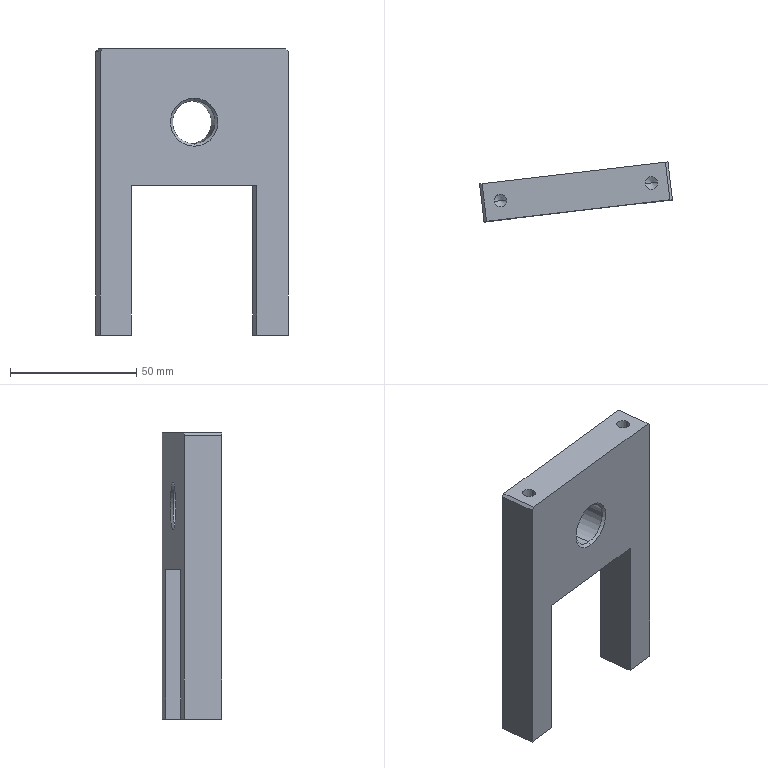Component | SolidWorks | 8TC-A17001-90-02PressureRollerSidePlate2-1 | 1 solid | 34 faces | box 76.24 x 23.65 x 113.2 mm | volume 77668 mm3 | cone 12 | plane 12 | cylinder 10 | commonest cylinder face diameters 5 x8 17 x2 | material #45
build123d program:
from build123d import *

# Parameters (mm, degrees)
SKETCH1_W                  = 75
SKETCH1_H                  = 54
BOSS_EXTRUDE1_DEPTH        = 7.5
SKETCH23_W                 = 12.5
SKETCH23_H                 = 15
BOSS_EXTRUDE4_DEPTH        = 59.2
M6_TAPPED_HOLE2_D          = 5
M6_TAPPED_HOLE2_DEPTH      = 25
M6_TAPPED_HOLE2_TIP        = 1.502
M6_TAPPED_HOLE1_D          = 5
M6_TAPPED_HOLE1_DEPTH      = 20
M6_TAPPED_HOLE1_TIP        = 1.502
F_15_0_15_DIAMETER_HOLE1_D = 17
CHAMFER2_SIZE              = 1


with BuildPart() as part:
    # Sketch1 → Boss-Extrude1 (new, symmetric)
    with BuildSketch(Plane(origin=(0, 0, 0), x_dir=(1, 0, 0), z_dir=(0, 1, 0))):
        Rectangle(SKETCH1_W, SKETCH1_H)
    extrude(amount=BOSS_EXTRUDE1_DEPTH, both=True)

    # Sketch23 → Boss-Extrude4 (add)
    with BuildSketch(Plane.XY.offset(27)):
        with Locations((-31.25, 0)):
            Rectangle(SKETCH23_W, SKETCH23_H)
        with Locations((31.25, 0)):
            Rectangle(SKETCH23_W, SKETCH23_H)
    extrude(amount=BOSS_EXTRUDE4_DEPTH)

    # M6 Tapped Hole2
    with Locations(Plane.XY.offset(86.2)):
        with Locations((-30, 0), (30, 0)):
            Hole(M6_TAPPED_HOLE2_D / 2, depth=M6_TAPPED_HOLE2_DEPTH)
            with Locations((0, 0, -(M6_TAPPED_HOLE2_DEPTH + M6_TAPPED_HOLE2_TIP / 2))):  # 118° drill point
                Cone(0, M6_TAPPED_HOLE2_D / 2, M6_TAPPED_HOLE2_TIP, mode=Mode.SUBTRACT)

    # M6 Tapped Hole1
    with Locations(Plane(origin=(0, 0, -27), x_dir=(-1, 0, 0), z_dir=(0, 0, -1))):
        with Locations((-30, 0), (30, 0)):
            Hole(M6_TAPPED_HOLE1_D / 2, depth=M6_TAPPED_HOLE1_DEPTH)
            with Locations((0, 0, -(M6_TAPPED_HOLE1_DEPTH + M6_TAPPED_HOLE1_TIP / 2))):  # 118° drill point
                Cone(0, M6_TAPPED_HOLE1_D / 2, M6_TAPPED_HOLE1_TIP, mode=Mode.SUBTRACT)

    # 15.0 _15_ Diameter Hole1 (through all)
    with Locations(Plane(origin=(0, 7.5, 0), x_dir=(1, 0, 0), z_dir=(0, 1, 0))):
        with Locations((0, -2)):
            Hole(F_15_0_15_DIAMETER_HOLE1_D / 2)

    # Chamfer2
    chamfer2_edges = [part.edges().sort_by_distance(p)[0] for p in [
        (8.5, -7.5, 2),
        (8.5, 7.5, 2),
        (-37.5, 0, -27),
        (37.5, 0, -27),
    ]]
    chamfer(chamfer2_edges, length=CHAMFER2_SIZE)


solid = part.part

# Placed as in the assembly
solid = solid.moved(Location((-0.2049, 42.224, -50), (180, 0, 173.3)))
STEP:
#1=COLOUR_RGB('',0.7922,0.8196,0.9333);
#2=FILL_AREA_STYLE_COLOUR('',#1);
#3=FILL_AREA_STYLE('',(#2));
#4=SURFACE_STYLE_FILL_AREA(#3);
#5=SURFACE_SIDE_STYLE('',(#4));
#6=SURFACE_STYLE_USAGE(.BOTH.,#5);
#7=PRESENTATION_STYLE_ASSIGNMENT((#6));
#8=CARTESIAN_POINT('',(-0.03792,1.917,-1.713));
#9=VERTEX_POINT('',#8);
#10=CARTESIAN_POINT('',(-0.03792,1.917,-2.382));
#11=VERTEX_POINT('',#10);
#12=CARTESIAN_POINT('',(-0.03792,1.917,-2.047));
#13=DIRECTION('',(-0.1167,0.9932,0.));
#14=DIRECTION('',(-0.,0.,-1.));
#15=AXIS2_PLACEMENT_3D('',#12,#13,#14);
#16=CIRCLE('',#15,0.3346);
#17=EDGE_CURVE('',#9,#11,#16,.T.);
#18=ORIENTED_EDGE('',*,*,#17,.F.);
#19=CARTESIAN_POINT('',(-0.04251,1.956,-1.673));
#20=VERTEX_POINT('',#19);
#21=CARTESIAN_POINT('',(-0.03792,1.917,-1.713));
#22=DIRECTION('',(-0.0825,0.7023,0.7071));
#23=VECTOR('',#22,39.37);
#24=LINE('',#21,#23);
#25=EDGE_CURVE('',#9,#20,#24,.T.);
#26=ORIENTED_EDGE('',*,*,#25,.T.);
#27=CARTESIAN_POINT('',(-0.04251,1.956,-2.421));
#28=VERTEX_POINT('',#27);
#29=CARTESIAN_POINT('',(-0.04251,1.956,-2.047));
#30=DIRECTION('',(0.1167,-0.9932,-0.));
#31=DIRECTION('',(-0.,0.,-1.));
#32=AXIS2_PLACEMENT_3D('',#29,#30,#31);
#33=CIRCLE('',#32,0.374);
#34=EDGE_CURVE('',#28,#20,#33,.T.);
#35=ORIENTED_EDGE('',*,*,#34,.F.);
#36=CARTESIAN_POINT('',(-0.03792,1.917,-2.382));
#37=DIRECTION('',(-0.0825,0.7023,-0.7071));
#38=VECTOR('',#37,39.37);
#39=LINE('',#36,#38);
#40=EDGE_CURVE('',#11,#28,#39,.T.);
#41=ORIENTED_EDGE('',*,*,#40,.F.);
#42=EDGE_LOOP('',(#18,#26,#35,#41));
#43=FACE_OUTER_BOUND('',#42,.T.);
#44=CARTESIAN_POINT('',(-0.03792,1.917,-2.047));
#45=DIRECTION('',(-0.1167,0.9932,0.));
#46=DIRECTION('',(-0.,0.,-1.));
#47=AXIS2_PLACEMENT_3D('',#44,#45,#46);
#48=CONICAL_SURFACE('',#47,0.3346,0.7854);
#49=ADVANCED_FACE('',(#43),#48,.F.);
#50=CARTESIAN_POINT('',(0.02179,1.408,-2.382));
#51=VERTEX_POINT('',#50);
#52=CARTESIAN_POINT('',(0.02179,1.408,-1.713));
#53=VERTEX_POINT('',#52);
#54=CARTESIAN_POINT('',(0.02179,1.408,-2.047));
#55=DIRECTION('',(0.1167,-0.9932,-0.));
#56=DIRECTION('',(-0.,0.,-1.));
#57=AXIS2_PLACEMENT_3D('',#54,#55,#56);
#58=CIRCLE('',#57,0.3346);
#59=EDGE_CURVE('',#51,#53,#58,.T.);
#60=ORIENTED_EDGE('',*,*,#59,.F.);
#61=CARTESIAN_POINT('',(0.02638,1.369,-2.421));
#62=VERTEX_POINT('',#61);
#63=CARTESIAN_POINT('',(0.02638,1.369,-2.421));
#64=DIRECTION('',(0.0825,-0.7023,-0.7071));
#65=VECTOR('',#64,39.37);
#66=LINE('',#63,#65);
#67=EDGE_CURVE('',#51,#62,#66,.T.);
#68=ORIENTED_EDGE('',*,*,#67,.T.);
#69=CARTESIAN_POINT('',(0.02638,1.369,-1.673));
#70=VERTEX_POINT('',#69);
#71=CARTESIAN_POINT('',(0.02638,1.369,-2.047));
#72=DIRECTION('',(-0.1167,0.9932,0.));
#73=DIRECTION('',(-0.,0.,-1.));
#74=AXIS2_PLACEMENT_3D('',#71,#72,#73);
#75=CIRCLE('',#74,0.374);
#76=EDGE_CURVE('',#70,#62,#75,.T.);
#77=ORIENTED_EDGE('',*,*,#76,.F.);
#78=CARTESIAN_POINT('',(0.02638,1.369,-1.673));
#79=DIRECTION('',(0.0825,-0.7023,0.7071));
#80=VECTOR('',#79,39.37);
#81=LINE('',#78,#80);
#82=EDGE_CURVE('',#53,#70,#81,.T.);
#83=ORIENTED_EDGE('',*,*,#82,.F.);
#84=EDGE_LOOP('',(#60,#68,#77,#83));
#85=FACE_OUTER_BOUND('',#84,.T.);
#86=CARTESIAN_POINT('',(0.02638,1.369,-2.047));
#87=DIRECTION('',(0.1167,-0.9932,-0.));
#88=DIRECTION('',(0.,0.,1.));
#89=AXIS2_PLACEMENT_3D('',#86,#87,#88);
#90=CONICAL_SURFACE('',#89,0.374,0.7854);
#91=ADVANCED_FACE('',(#85),#90,.F.);
#92=ORIENTED_EDGE('',*,*,#59,.T.);
#93=CARTESIAN_POINT('',(-0.04251,1.956,-1.713));
#94=DIRECTION('',(-0.1167,0.9932,0.));
#95=VECTOR('',#94,39.37);
#96=LINE('',#93,#95);
#97=EDGE_CURVE('',#53,#9,#96,.T.);
#98=ORIENTED_EDGE('',*,*,#97,.T.);
#99=ORIENTED_EDGE('',*,*,#17,.T.);
#100=CARTESIAN_POINT('',(-0.04251,1.956,-2.382));
#101=DIRECTION('',(-0.1167,0.9932,0.));
#102=VECTOR('',#101,39.37);
#103=LINE('',#100,#102);
#104=EDGE_CURVE('',#51,#11,#103,.T.);
#105=ORIENTED_EDGE('',*,*,#104,.F.);
#106=EDGE_LOOP('',(#92,#98,#99,#105));
#107=FACE_OUTER_BOUND('',#106,.T.);
#108=CARTESIAN_POINT('',(-0.04251,1.956,-2.047));
#109=DIRECTION('',(-0.1167,0.9932,0.));
#110=DIRECTION('',(-0.,0.,-1.));
#111=AXIS2_PLACEMENT_3D('',#108,#109,#110);
#112=CYLINDRICAL_SURFACE('',#111,0.3346);
#113=ADVANCED_FACE('',(#107),#112,.F.);
#114=CARTESIAN_POINT('',(-1.279,1.513,-1.693));
#115=VERTEX_POINT('',#114);
#116=CARTESIAN_POINT('',(-1.083,1.536,-1.693));
#117=VERTEX_POINT('',#116);
#118=CARTESIAN_POINT('',(-1.181,1.525,-1.693));
#119=DIRECTION('',(0.,-0.,1.));
#120=DIRECTION('',(0.9932,0.1167,0.));
#121=AXIS2_PLACEMENT_3D('',#118,#119,#120);
#122=CIRCLE('',#121,0.09843);
#123=EDGE_CURVE('',#115,#117,#122,.T.);
#124=ORIENTED_EDGE('',*,*,#123,.F.);
#125=CARTESIAN_POINT('',(-1.279,1.513,-0.9055));
#126=VERTEX_POINT('',#125);
#127=CARTESIAN_POINT('',(-1.279,1.513,-0.9055));
#128=DIRECTION('',(0.,-0.,1.));
#129=VECTOR('',#128,39.37);
#130=LINE('',#127,#129);
#131=EDGE_CURVE('',#115,#126,#130,.T.);
#132=ORIENTED_EDGE('',*,*,#131,.T.);
#133=CARTESIAN_POINT('',(-1.083,1.536,-0.9055));
#134=VERTEX_POINT('',#133);
#135=CARTESIAN_POINT('',(-1.181,1.525,-0.9055));
#136=DIRECTION('',(0.,-0.,1.));
#137=DIRECTION('',(0.9932,0.1167,0.));
#138=AXIS2_PLACEMENT_3D('',#135,#136,#137);
#139=CIRCLE('',#138,0.09843);
#140=EDGE_CURVE('',#126,#134,#139,.T.);
#141=ORIENTED_EDGE('',*,*,#140,.T.);
#142=CARTESIAN_POINT('',(-1.083,1.536,-0.9055));
#143=DIRECTION('',(0.,-0.,1.));
#144=VECTOR('',#143,39.37);
#145=LINE('',#142,#144);
#146=EDGE_CURVE('',#117,#134,#145,.T.);
#147=ORIENTED_EDGE('',*,*,#146,.F.);
#148=EDGE_LOOP('',(#124,#132,#141,#147));
#149=FACE_OUTER_BOUND('',#148,.T.);
#150=CARTESIAN_POINT('',(-1.181,1.525,-0.9055));
#151=DIRECTION('',(0.,-0.,1.));
#152=DIRECTION('',(0.9932,0.1167,0.));
#153=AXIS2_PLACEMENT_3D('',#150,#151,#152);
#154=CYLINDRICAL_SURFACE('',#153,0.09843);
#155=ADVANCED_FACE('',(#149),#154,.F.);
#156=CARTESIAN_POINT('',(-1.181,1.525,-1.752));
#157=VERTEX_POINT('',#156);
#158=CARTESIAN_POINT('',(-1.083,1.536,-1.693));
#159=DIRECTION('',(0.8513,0.1,0.515));
#160=VECTOR('',#159,39.37);
#161=LINE('',#158,#160);
#162=EDGE_CURVE('',#157,#117,#161,.T.);
#163=ORIENTED_EDGE('',*,*,#162,.F.);
#164=CARTESIAN_POINT('',(-1.279,1.513,-1.693));
#165=DIRECTION('',(-0.8513,-0.1,0.515));
#166=VECTOR('',#165,39.37);
#167=LINE('',#164,#166);
#168=EDGE_CURVE('',#157,#115,#167,.T.);
#169=ORIENTED_EDGE('',*,*,#168,.T.);
#170=ORIENTED_EDGE('',*,*,#123,.T.);
#171=EDGE_LOOP('',(#163,#169,#170));
#172=FACE_OUTER_BOUND('',#171,.T.);
#173=CARTESIAN_POINT('',(-1.181,1.525,-1.693));
#174=DIRECTION('',(0.,-0.,1.));
#175=DIRECTION('',(0.9932,0.1167,0.));
#176=AXIS2_PLACEMENT_3D('',#173,#174,#175);
#177=CONICAL_SURFACE('',#176,0.09843,1.03);
#178=ADVANCED_FACE('',(#172),#177,.F.);
#179=CARTESIAN_POINT('',(1.067,1.789,-1.693));
#180=VERTEX_POINT('',#179);
#181=CARTESIAN_POINT('',(1.263,1.812,-1.693));
#182=VERTEX_POINT('',#181);
#183=CARTESIAN_POINT('',(1.165,1.8,-1.693));
#184=DIRECTION('',(0.,-0.,1.));
#185=DIRECTION('',(0.9932,0.1167,0.));
#186=AXIS2_PLACEMENT_3D('',#183,#184,#185);
#187=CIRCLE('',#186,0.09843);
#188=EDGE_CURVE('',#180,#182,#187,.T.);
#189=ORIENTED_EDGE('',*,*,#188,.F.);
#190=CARTESIAN_POINT('',(1.067,1.789,-0.9055));
#191=VERTEX_POINT('',#190);
#192=CARTESIAN_POINT('',(1.067,1.789,-0.9055));
#193=DIRECTION('',(0.,-0.,1.));
#194=VECTOR('',#193,39.37);
#195=LINE('',#192,#194);
#196=EDGE_CURVE('',#180,#191,#195,.T.);
#197=ORIENTED_EDGE('',*,*,#196,.T.);
#198=CARTESIAN_POINT('',(1.263,1.812,-0.9055));
#199=VERTEX_POINT('',#198);
#200=CARTESIAN_POINT('',(1.165,1.8,-0.9055));
#201=DIRECTION('',(0.,-0.,1.));
#202=DIRECTION('',(0.9932,0.1167,0.));
#203=AXIS2_PLACEMENT_3D('',#200,#201,#202);
#204=CIRCLE('',#203,0.09843);
#205=EDGE_CURVE('',#191,#199,#204,.T.);
#206=ORIENTED_EDGE('',*,*,#205,.T.);
#207=CARTESIAN_POINT('',(1.263,1.812,-0.9055));
#208=DIRECTION('',(0.,-0.,1.));
#209=VECTOR('',#208,39.37);
#210=LINE('',#207,#209);
#211=EDGE_CURVE('',#182,#199,#210,.T.);
#212=ORIENTED_EDGE('',*,*,#211,.F.);
#213=EDGE_LOOP('',(#189,#197,#206,#212));
#214=FACE_OUTER_BOUND('',#213,.T.);
#215=CARTESIAN_POINT('',(1.165,1.8,-0.9055));
#216=DIRECTION('',(0.,-0.,1.));
#217=DIRECTION('',(0.9932,0.1167,0.));
#218=AXIS2_PLACEMENT_3D('',#215,#216,#217);
#219=CYLINDRICAL_SURFACE('',#218,0.09843);
#220=ADVANCED_FACE('',(#214),#219,.F.);
#221=CARTESIAN_POINT('',(1.165,1.8,-1.752));
#222=VERTEX_POINT('',#221);
#223=CARTESIAN_POINT('',(1.263,1.812,-1.693));
#224=DIRECTION('',(0.8513,0.1,0.515));
#225=VECTOR('',#224,39.37);
#226=LINE('',#223,#225);
#227=EDGE_CURVE('',#222,#182,#226,.T.);
#228=ORIENTED_EDGE('',*,*,#227,.F.);
#229=CARTESIAN_POINT('',(1.067,1.789,-1.693));
#230=DIRECTION('',(-0.8513,-0.1,0.515));
#231=VECTOR('',#230,39.37);
#232=LINE('',#229,#231);
#233=EDGE_CURVE('',#222,#180,#232,.T.);
#234=ORIENTED_EDGE('',*,*,#233,.T.);
#235=ORIENTED_EDGE('',*,*,#188,.T.);
#236=EDGE_LOOP('',(#228,#234,#235));
#237=FACE_OUTER_BOUND('',#236,.T.);
#238=CARTESIAN_POINT('',(1.165,1.8,-1.693));
#239=DIRECTION('',(0.,-0.,1.));
#240=DIRECTION('',(0.9932,0.1167,0.));
#241=AXIS2_PLACEMENT_3D('',#238,#239,#240);
#242=CONICAL_SURFACE('',#241,0.09843,1.03);
#243=ADVANCED_FACE('',(#237),#242,.F.);
#244=CARTESIAN_POINT('',(1.263,1.812,-4.378));
#245=VERTEX_POINT('',#244);
#246=CARTESIAN_POINT('',(1.067,1.789,-4.378));
#247=VERTEX_POINT('',#246);
#248=CARTESIAN_POINT('',(1.165,1.8,-4.378));
#249=DIRECTION('',(-0.,0.,-1.));
#250=DIRECTION('',(-0.9932,-0.1167,0.));
#251=AXIS2_PLACEMENT_3D('',#248,#249,#250);
#252=CIRCLE('',#251,0.09843);
#253=EDGE_CURVE('',#245,#247,#252,.T.);
#254=ORIENTED_EDGE('',*,*,#253,.F.);
#255=CARTESIAN_POINT('',(1.263,1.812,-5.362));
#256=VERTEX_POINT('',#255);
#257=CARTESIAN_POINT('',(1.263,1.812,-5.362));
#258=DIRECTION('',(-0.,0.,-1.));
#259=VECTOR('',#258,39.37);
#260=LINE('',#257,#259);
#261=EDGE_CURVE('',#245,#256,#260,.T.);
#262=ORIENTED_EDGE('',*,*,#261,.T.);
#263=CARTESIAN_POINT('',(1.067,1.789,-5.362));
#264=VERTEX_POINT('',#263);
#265=CARTESIAN_POINT('',(1.165,1.8,-5.362));
#266=DIRECTION('',(-0.,0.,-1.));
#267=DIRECTION('',(-0.9932,-0.1167,0.));
#268=AXIS2_PLACEMENT_3D('',#265,#266,#267);
#269=CIRCLE('',#268,0.09843);
#270=EDGE_CURVE('',#256,#264,#269,.T.);
#271=ORIENTED_EDGE('',*,*,#270,.T.);
#272=CARTESIAN_POINT('',(1.067,1.789,-5.362));
#273=DIRECTION('',(-0.,0.,-1.));
#274=VECTOR('',#273,39.37);
#275=LINE('',#272,#274);
#276=EDGE_CURVE('',#247,#264,#275,.T.);
#277=ORIENTED_EDGE('',*,*,#276,.F.);
#278=EDGE_LOOP('',(#254,#262,#271,#277));
#279=FACE_OUTER_BOUND('',#278,.T.);
#280=CARTESIAN_POINT('',(1.165,1.8,-5.362));
#281=DIRECTION('',(-0.,0.,-1.));
#282=DIRECTION('',(-0.9932,-0.1167,0.));
#283=AXIS2_PLACEMENT_3D('',#280,#281,#282);
#284=CYLINDRICAL_SURFACE('',#283,0.09843);
#285=ADVANCED_FACE('',(#279),#284,.F.);
#286=CARTESIAN_POINT('',(1.165,1.8,-4.319));
#287=VERTEX_POINT('',#286);
#288=CARTESIAN_POINT('',(1.067,1.789,-4.378));
#289=DIRECTION('',(-0.8513,-0.1,-0.515));
#290=VECTOR('',#289,39.37);
#291=LINE('',#288,#290);
#292=EDGE_CURVE('',#287,#247,#291,.T.);
#293=ORIENTED_EDGE('',*,*,#292,.F.);
#294=CARTESIAN_POINT('',(1.263,1.812,-4.378));
#295=DIRECTION('',(0.8513,0.1,-0.515));
#296=VECTOR('',#295,39.37);
#297=LINE('',#294,#296);
#298=EDGE_CURVE('',#287,#245,#297,.T.);
#299=ORIENTED_EDGE('',*,*,#298,.T.);
#300=ORIENTED_EDGE('',*,*,#253,.T.);
#301=EDGE_LOOP('',(#293,#299,#300));
#302=FACE_OUTER_BOUND('',#301,.T.);
#303=CARTESIAN_POINT('',(1.165,1.8,-4.378));
#304=DIRECTION('',(-0.,0.,-1.));
#305=DIRECTION('',(-0.9932,-0.1167,0.));
#306=AXIS2_PLACEMENT_3D('',#303,#304,#305);
#307=CONICAL_SURFACE('',#306,0.09843,1.03);
#308=ADVANCED_FACE('',(#302),#307,.F.);
#309=CARTESIAN_POINT('',(-1.083,1.536,-4.378));
#310=VERTEX_POINT('',#309);
#311=CARTESIAN_POINT('',(-1.279,1.513,-4.378));
#312=VERTEX_POINT('',#311);
#313=CARTESIAN_POINT('',(-1.181,1.525,-4.378));
#314=DIRECTION('',(-0.,0.,-1.));
#315=DIRECTION('',(-0.9932,-0.1167,0.));
#316=AXIS2_PLACEMENT_3D('',#313,#314,#315);
#317=CIRCLE('',#316,0.09843);
#318=EDGE_CURVE('',#310,#312,#317,.T.);
#319=ORIENTED_EDGE('',*,*,#318,.F.);
#320=CARTESIAN_POINT('',(-1.083,1.536,-5.362));
#321=VERTEX_POINT('',#320);
#322=CARTESIAN_POINT('',(-1.083,1.536,-5.362));
#323=DIRECTION('',(-0.,0.,-1.));
#324=VECTOR('',#323,39.37);
#325=LINE('',#322,#324);
#326=EDGE_CURVE('',#310,#321,#325,.T.);
#327=ORIENTED_EDGE('',*,*,#326,.T.);
#328=CARTESIAN_POINT('',(-1.279,1.513,-5.362));
#329=VERTEX_POINT('',#328);
#330=CARTESIAN_POINT('',(-1.181,1.525,-5.362));
#331=DIRECTION('',(-0.,0.,-1.));
#332=DIRECTION('',(-0.9932,-0.1167,0.));
#333=AXIS2_PLACEMENT_3D('',#330,#331,#332);
#334=CIRCLE('',#333,0.09843);
#335=EDGE_CURVE('',#321,#329,#334,.T.);
#336=ORIENTED_EDGE('',*,*,#335,.T.);
#337=CARTESIAN_POINT('',(-1.279,1.513,-5.362));
#338=DIRECTION('',(-0.,0.,-1.));
#339=VECTOR('',#338,39.37);
#340=LINE('',#337,#339);
#341=EDGE_CURVE('',#312,#329,#340,.T.);
#342=ORIENTED_EDGE('',*,*,#341,.F.);
#343=EDGE_LOOP('',(#319,#327,#336,#342));
#344=FACE_OUTER_BOUND('',#343,.T.);
#345=CARTESIAN_POINT('',(-1.181,1.525,-5.362));
#346=DIRECTION('',(-0.,0.,-1.));
#347=DIRECTION('',(-0.9932,-0.1167,0.));
#348=AXIS2_PLACEMENT_3D('',#345,#346,#347);
#349=CYLINDRICAL_SURFACE('',#348,0.09843);
#350=ADVANCED_FACE('',(#344),#349,.F.);
#351=CARTESIAN_POINT('',(-1.181,1.525,-4.319));
#352=VERTEX_POINT('',#351);
#353=CARTESIAN_POINT('',(-1.279,1.513,-4.378));
#354=DIRECTION('',(-0.8513,-0.1,-0.515));
#355=VECTOR('',#354,39.37);
#356=LINE('',#353,#355);
#357=EDGE_CURVE('',#352,#312,#356,.T.);
#358=ORIENTED_EDGE('',*,*,#357,.F.);
#359=CARTESIAN_POINT('',(-1.083,1.536,-4.378));
#360=DIRECTION('',(0.8513,0.1,-0.515));
#361=VECTOR('',#360,39.37);
#362=LINE('',#359,#361);
#363=EDGE_CURVE('',#352,#310,#362,.T.);
#364=ORIENTED_EDGE('',*,*,#363,.T.);
#365=ORIENTED_EDGE('',*,*,#318,.T.);
#366=EDGE_LOOP('',(#358,#364,#365));
#367=FACE_OUTER_BOUND('',#366,.T.);
#368=CARTESIAN_POINT('',(-1.181,1.525,-4.378));
#369=DIRECTION('',(-0.,0.,-1.));
#370=DIRECTION('',(-0.9932,-0.1167,0.));
#371=AXIS2_PLACEMENT_3D('',#368,#369,#370);
#372=CONICAL_SURFACE('',#371,0.09843,1.03);
#373=ADVANCED_FACE('',(#367),#372,.F.);
#374=CARTESIAN_POINT('',(-1.02,1.841,-3.031));
#375=VERTEX_POINT('',#374);
#376=CARTESIAN_POINT('',(-0.9511,1.254,-3.031));
#377=VERTEX_POINT('',#376);
#378=CARTESIAN_POINT('',(-1.02,1.841,-3.031));
#379=DIRECTION('',(0.1167,-0.9932,-0.));
#380=VECTOR('',#379,39.37);
#381=LINE('',#378,#380);
#382=EDGE_CURVE('',#375,#377,#381,.T.);
#383=ORIENTED_EDGE('',*,*,#382,.F.);
#384=CARTESIAN_POINT('',(0.935,2.07,-3.031));
#385=VERTEX_POINT('',#384);
#386=CARTESIAN_POINT('',(1.424,2.128,-3.031));
#387=DIRECTION('',(-0.9932,-0.1167,0.));
#388=VECTOR('',#387,39.37);
#389=LINE('',#386,#388);
#390=EDGE_CURVE('',#385,#375,#389,.T.);
#391=ORIENTED_EDGE('',*,*,#390,.F.);
#392=CARTESIAN_POINT('',(1.004,1.484,-3.031));
#393=VERTEX_POINT('',#392);
#394=CARTESIAN_POINT('',(0.935,2.07,-3.031));
#395=DIRECTION('',(-0.1167,0.9932,0.));
#396=VECTOR('',#395,39.37);
#397=LINE('',#394,#396);
#398=EDGE_CURVE('',#393,#385,#397,.T.);
#399=ORIENTED_EDGE('',*,*,#398,.F.);
#400=CARTESIAN_POINT('',(1.493,1.541,-3.031));
#401=DIRECTION('',(-0.9932,-0.1167,0.));
#402=VECTOR('',#401,39.37);
#403=LINE('',#400,#402);
#404=EDGE_CURVE('',#393,#377,#403,.T.);
#405=ORIENTED_EDGE('',*,*,#404,.T.);
#406=EDGE_LOOP('',(#383,#391,#399,#405));
#407=FACE_OUTER_BOUND('',#406,.T.);
#408=CARTESIAN_POINT('',(1.424,2.128,-3.031));
#409=DIRECTION('',(0.,-0.,1.));
#410=DIRECTION('',(0.9932,0.1167,-0.));
#411=AXIS2_PLACEMENT_3D('',#408,#409,#410);
#412=PLANE('',#411);
#413=ADVANCED_FACE('',(#407),#412,.F.);
#414=CARTESIAN_POINT('',(-1.44,1.197,-5.362));
#415=VERTEX_POINT('',#414);
#416=CARTESIAN_POINT('',(-1.44,1.197,-0.9449));
#417=VERTEX_POINT('',#416);
#418=CARTESIAN_POINT('',(-1.44,1.197,-0.9055));
#419=DIRECTION('',(0.,-0.,1.));
#420=VECTOR('',#419,39.37);
#421=LINE('',#418,#420);
#422=EDGE_CURVE('',#415,#417,#421,.T.);
#423=ORIENTED_EDGE('',*,*,#422,.T.);
#424=CARTESIAN_POINT('',(-1.509,1.783,-0.9449));
#425=VERTEX_POINT('',#424);
#426=CARTESIAN_POINT('',(-1.509,1.783,-0.9449));
#427=DIRECTION('',(-0.1167,0.9932,0.));
#428=VECTOR('',#427,39.37);
#429=LINE('',#426,#428);
#430=EDGE_CURVE('',#417,#425,#429,.T.);
#431=ORIENTED_EDGE('',*,*,#430,.T.);
#432=CARTESIAN_POINT('',(-1.509,1.783,-5.362));
#433=VERTEX_POINT('',#432);
#434=CARTESIAN_POINT('',(-1.509,1.783,-0.9055));
#435=DIRECTION('',(0.,-0.,1.));
#436=VECTOR('',#435,39.37);
#437=LINE('',#434,#436);
#438=EDGE_CURVE('',#433,#425,#437,.T.);
#439=ORIENTED_EDGE('',*,*,#438,.F.);
#440=CARTESIAN_POINT('',(-1.509,1.783,-5.362));
#441=DIRECTION('',(-0.1167,0.9932,0.));
#442=VECTOR('',#441,39.37);
#443=LINE('',#440,#442);
#444=EDGE_CURVE('',#415,#433,#443,.T.);
#445=ORIENTED_EDGE('',*,*,#444,.F.);
#446=EDGE_LOOP('',(#423,#431,#439,#445));
#447=FACE_OUTER_BOUND('',#446,.T.);
#448=CARTESIAN_POINT('',(-1.509,1.783,-0.9055));
#449=DIRECTION('',(0.9932,0.1167,-0.));
#450=DIRECTION('',(-0.,0.,-1.));
#451=AXIS2_PLACEMENT_3D('',#448,#449,#450);
#452=PLANE('',#451);
#453=ADVANCED_FACE('',(#447),#452,.F.);
#454=CARTESIAN_POINT('',(-1.181,1.525,-0.9055));
#455=DIRECTION('',(0.,-0.,1.));
#456=DIRECTION('',(0.9932,0.1167,0.));
#457=AXIS2_PLACEMENT_3D('',#454,#455,#456);
#458=CIRCLE('',#457,0.09843);
#459=EDGE_CURVE('',#134,#126,#458,.T.);
#460=ORIENTED_EDGE('',*,*,#459,.F.);
#461=ORIENTED_EDGE('',*,*,#140,.F.);
#462=EDGE_LOOP('',(#460,#461));
#463=FACE_BOUND('',#462,.T.);
#464=CARTESIAN_POINT('',(1.165,1.8,-0.9055));
#465=DIRECTION('',(0.,-0.,1.));
#466=DIRECTION('',(0.9932,0.1167,0.));
#467=AXIS2_PLACEMENT_3D('',#464,#465,#466);
#468=CIRCLE('',#467,0.09843);
#469=EDGE_CURVE('',#199,#191,#468,.T.);
#470=ORIENTED_EDGE('',*,*,#469,.F.);
#471=ORIENTED_EDGE('',*,*,#205,.F.);
#472=EDGE_LOOP('',(#470,#471));
#473=FACE_BOUND('',#472,.T.);
#474=CARTESIAN_POINT('',(-1.401,1.201,-0.9055));
#475=VERTEX_POINT('',#474);
#476=CARTESIAN_POINT('',(1.454,1.537,-0.9055));
#477=VERTEX_POINT('',#476);
#478=CARTESIAN_POINT('',(1.493,1.541,-0.9055));
#479=DIRECTION('',(0.9932,0.1167,-0.));
#480=VECTOR('',#479,39.37);
#481=LINE('',#478,#480);
#482=EDGE_CURVE('',#475,#477,#481,.T.);
#483=ORIENTED_EDGE('',*,*,#482,.T.);
#484=CARTESIAN_POINT('',(1.385,2.123,-0.9055));
#485=VERTEX_POINT('',#484);
#486=CARTESIAN_POINT('',(1.385,2.123,-0.9055));
#487=DIRECTION('',(-0.1167,0.9932,0.));
#488=VECTOR('',#487,39.37);
#489=LINE('',#486,#488);
#490=EDGE_CURVE('',#477,#485,#489,.T.);
#491=ORIENTED_EDGE('',*,*,#490,.T.);
#492=CARTESIAN_POINT('',(-1.47,1.788,-0.9055));
#493=VERTEX_POINT('',#492);
#494=CARTESIAN_POINT('',(1.424,2.128,-0.9055));
#495=DIRECTION('',(0.9932,0.1167,-0.));
#496=VECTOR('',#495,39.37);
#497=LINE('',#494,#496);
#498=EDGE_CURVE('',#493,#485,#497,.T.);
#499=ORIENTED_EDGE('',*,*,#498,.F.);
#500=CARTESIAN_POINT('',(-1.47,1.788,-0.9055));
#501=DIRECTION('',(0.1167,-0.9932,-0.));
#502=VECTOR('',#501,39.37);
#503=LINE('',#500,#502);
#504=EDGE_CURVE('',#493,#475,#503,.T.);
#505=ORIENTED_EDGE('',*,*,#504,.T.);
#506=EDGE_LOOP('',(#483,#491,#499,#505));
#507=FACE_OUTER_BOUND('',#506,.T.);
#508=CARTESIAN_POINT('',(1.424,2.128,-0.9055));
#509=DIRECTION('',(-0.,0.,-1.));
#510=DIRECTION('',(-0.9932,-0.1167,0.));
#511=AXIS2_PLACEMENT_3D('',#508,#509,#510);
#512=PLANE('',#511);
#513=ADVANCED_FACE('',(#463,#473,#507),#512,.F.);
#514=CARTESIAN_POINT('',(1.424,2.128,-0.9449));
#515=VERTEX_POINT('',#514);
#516=CARTESIAN_POINT('',(1.424,2.128,-5.362));
#517=VERTEX_POINT('',#516);
#518=CARTESIAN_POINT('',(1.424,2.128,-0.9055));
#519=DIRECTION('',(-0.,0.,-1.));
#520=VECTOR('',#519,39.37);
#521=LINE('',#518,#520);
#522=EDGE_CURVE('',#515,#517,#521,.T.);
#523=ORIENTED_EDGE('',*,*,#522,.F.);
#524=CARTESIAN_POINT('',(1.493,1.541,-0.9449));
#525=VERTEX_POINT('',#524);
#526=CARTESIAN_POINT('',(1.424,2.128,-0.9449));
#527=DIRECTION('',(0.1167,-0.9932,-0.));
#528=VECTOR('',#527,39.37);
#529=LINE('',#526,#528);
#530=EDGE_CURVE('',#515,#525,#529,.T.);
#531=ORIENTED_EDGE('',*,*,#530,.T.);
#532=CARTESIAN_POINT('',(1.493,1.541,-5.362));
#533=VERTEX_POINT('',#532);
#534=CARTESIAN_POINT('',(1.493,1.541,-0.9055));
#535=DIRECTION('',(-0.,0.,-1.));
#536=VECTOR('',#535,39.37);
#537=LINE('',#534,#536);
#538=EDGE_CURVE('',#525,#533,#537,.T.);
#539=ORIENTED_EDGE('',*,*,#538,.T.);
#540=CARTESIAN_POINT('',(1.424,2.128,-5.362));
#541=DIRECTION('',(0.1167,-0.9932,-0.));
#542=VECTOR('',#541,39.37);
#543=LINE('',#540,#542);
#544=EDGE_CURVE('',#517,#533,#543,.T.);
#545=ORIENTED_EDGE('',*,*,#544,.F.);
#546=EDGE_LOOP('',(#523,#531,#539,#545));
#547=FACE_OUTER_BOUND('',#546,.T.);
#548=CARTESIAN_POINT('',(1.424,2.128,-0.9055));
#549=DIRECTION('',(-0.9932,-0.1167,0.));
#550=DIRECTION('',(0.,-0.,1.));
#551=AXIS2_PLACEMENT_3D('',#548,#549,#550);
#552=PLANE('',#551);
#553=ADVANCED_FACE('',(#547),#552,.F.);
#554=ORIENTED_EDGE('',*,*,#34,.T.);
#555=CARTESIAN_POINT('',(-0.04251,1.956,-2.047));
#556=DIRECTION('',(0.1167,-0.9932,-0.));
#557=DIRECTION('',(-0.,0.,-1.));
#558=AXIS2_PLACEMENT_3D('',#555,#556,#557);
#559=CIRCLE('',#558,0.374);
#560=EDGE_CURVE('',#20,#28,#559,.T.);
#561=ORIENTED_EDGE('',*,*,#560,.T.);
#562=EDGE_LOOP('',(#554,#561));
#563=FACE_BOUND('',#562,.T.);
#564=ORIENTED_EDGE('',*,*,#498,.T.);
#565=CARTESIAN_POINT('',(1.199,2.101,-0.7185));
#566=DIRECTION('',(0.7023,0.0825,-0.7071));
#567=VECTOR('',#566,39.37);
#568=LINE('',#565,#567);
#569=EDGE_CURVE('',#485,#515,#568,.T.);
#570=ORIENTED_EDGE('',*,*,#569,.T.);
#571=ORIENTED_EDGE('',*,*,#522,.T.);
#572=CARTESIAN_POINT('',(0.935,2.07,-5.362));
#573=VERTEX_POINT('',#572);
#574=CARTESIAN_POINT('',(1.424,2.128,-5.362));
#575=DIRECTION('',(0.9932,0.1167,-0.));
#576=VECTOR('',#575,39.37);
#577=LINE('',#574,#576);
#578=EDGE_CURVE('',#573,#517,#577,.T.);
#579=ORIENTED_EDGE('',*,*,#578,.F.);
#580=CARTESIAN_POINT('',(0.935,2.07,-5.362));
#581=DIRECTION('',(0.,-0.,1.));
#582=VECTOR('',#581,39.37);
#583=LINE('',#580,#582);
#584=EDGE_CURVE('',#573,#385,#583,.T.);
#585=ORIENTED_EDGE('',*,*,#584,.T.);
#586=ORIENTED_EDGE('',*,*,#390,.T.);
#587=CARTESIAN_POINT('',(-1.02,1.841,-5.362));
#588=VERTEX_POINT('',#587);
#589=CARTESIAN_POINT('',(-1.02,1.841,-5.362));
#590=DIRECTION('',(0.,-0.,1.));
#591=VECTOR('',#590,39.37);
#592=LINE('',#589,#591);
#593=EDGE_CURVE('',#588,#375,#592,.T.);
#594=ORIENTED_EDGE('',*,*,#593,.F.);
#595=CARTESIAN_POINT('',(-1.509,1.783,-5.362));
#596=DIRECTION('',(0.9932,0.1167,-0.));
#597=VECTOR('',#596,39.37);
#598=LINE('',#595,#597);
#599=EDGE_CURVE('',#433,#588,#598,.T.);
#600=ORIENTED_EDGE('',*,*,#599,.F.);
#601=ORIENTED_EDGE('',*,*,#438,.T.);
#602=CARTESIAN_POINT('',(-1.284,1.81,-0.7185));
#603=DIRECTION('',(0.7023,0.0825,0.7071));
#604=VECTOR('',#603,39.37);
#605=LINE('',#602,#604);
#606=EDGE_CURVE('',#425,#493,#605,.T.);
#607=ORIENTED_EDGE('',*,*,#606,.T.);
#608=EDGE_LOOP('',(#564,#570,#571,#579,#585,#586,#594,#600,#601,#607));
#609=FACE_OUTER_BOUND('',#608,.T.);
#610=CARTESIAN_POINT('',(-0.04251,1.956,-1.969));
#611=DIRECTION('',(-0.1167,0.9932,0.));
#612=DIRECTION('',(-0.,0.,-1.));
#613=AXIS2_PLACEMENT_3D('',#610,#611,#612);
#614=PLANE('',#613);
#615=ADVANCED_FACE('',(#563,#609),#614,.T.);
#616=ORIENTED_EDGE('',*,*,#76,.T.);
#617=CARTESIAN_POINT('',(0.02638,1.369,-2.047));
#618=DIRECTION('',(-0.1167,0.9932,0.));
#619=DIRECTION('',(-0.,0.,-1.));
#620=AXIS2_PLACEMENT_3D('',#617,#618,#619);
#621=CIRCLE('',#620,0.374);
#622=EDGE_CURVE('',#62,#70,#621,.T.);
#623=ORIENTED_EDGE('',*,*,#622,.T.);
#624=EDGE_LOOP('',(#616,#623));
#625=FACE_BOUND('',#624,.T.);
#626=ORIENTED_EDGE('',*,*,#538,.F.);
#627=CARTESIAN_POINT('',(1.493,1.541,-0.9449));
#628=DIRECTION('',(-0.7023,-0.0825,0.7071));
#629=VECTOR('',#628,39.37);
#630=LINE('',#627,#629);
#631=EDGE_CURVE('',#525,#477,#630,.T.);
#632=ORIENTED_EDGE('',*,*,#631,.T.);
#633=ORIENTED_EDGE('',*,*,#482,.F.);
#634=CARTESIAN_POINT('',(-1.401,1.201,-0.9055));
#635=DIRECTION('',(-0.7023,-0.0825,-0.7071));
#636=VECTOR('',#635,39.37);
#637=LINE('',#634,#636);
#638=EDGE_CURVE('',#475,#417,#637,.T.);
#639=ORIENTED_EDGE('',*,*,#638,.T.);
#640=ORIENTED_EDGE('',*,*,#422,.F.);
#641=CARTESIAN_POINT('',(-0.9511,1.254,-5.362));
#642=VERTEX_POINT('',#641);
#643=CARTESIAN_POINT('',(-1.44,1.197,-5.362));
#644=DIRECTION('',(-0.9932,-0.1167,0.));
#645=VECTOR('',#644,39.37);
#646=LINE('',#643,#645);
#647=EDGE_CURVE('',#642,#415,#646,.T.);
#648=ORIENTED_EDGE('',*,*,#647,.F.);
#649=CARTESIAN_POINT('',(-0.9511,1.254,-5.362));
#650=DIRECTION('',(0.,-0.,1.));
#651=VECTOR('',#650,39.37);
#652=LINE('',#649,#651);
#653=EDGE_CURVE('',#642,#377,#652,.T.);
#654=ORIENTED_EDGE('',*,*,#653,.T.);
#655=ORIENTED_EDGE('',*,*,#404,.F.);
#656=CARTESIAN_POINT('',(1.004,1.484,-5.362));
#657=VERTEX_POINT('',#656);
#658=CARTESIAN_POINT('',(1.004,1.484,-5.362));
#659=DIRECTION('',(0.,-0.,1.));
#660=VECTOR('',#659,39.37);
#661=LINE('',#658,#660);
#662=EDGE_CURVE('',#657,#393,#661,.T.);
#663=ORIENTED_EDGE('',*,*,#662,.F.);
#664=CARTESIAN_POINT('',(1.493,1.541,-5.362));
#665=DIRECTION('',(-0.9932,-0.1167,0.));
#666=VECTOR('',#665,39.37);
#667=LINE('',#664,#666);
#668=EDGE_CURVE('',#533,#657,#667,.T.);
#669=ORIENTED_EDGE('',*,*,#668,.F.);
#670=EDGE_LOOP('',(#626,#632,#633,#639,#640,#648,#654,#655,#663,#669));
#671=FACE_OUTER_BOUND('',#670,.T.);
#672=CARTESIAN_POINT('',(0.02638,1.369,-1.969));
#673=DIRECTION('',(-0.1167,0.9932,0.));
#674=DIRECTION('',(-0.,0.,-1.));
#675=AXIS2_PLACEMENT_3D('',#672,#673,#674);
#676=PLANE('',#675);
#677=ADVANCED_FACE('',(#625,#671),#676,.F.);
#678=ORIENTED_EDGE('',*,*,#398,.T.);
#679=ORIENTED_EDGE('',*,*,#584,.F.);
#680=CARTESIAN_POINT('',(0.935,2.07,-5.362));
#681=DIRECTION('',(-0.1167,0.9932,0.));
#682=VECTOR('',#681,39.37);
#683=LINE('',#680,#682);
#684=EDGE_CURVE('',#657,#573,#683,.T.);
#685=ORIENTED_EDGE('',*,*,#684,.F.);
#686=ORIENTED_EDGE('',*,*,#662,.T.);
#687=EDGE_LOOP('',(#678,#679,#685,#686));
#688=FACE_OUTER_BOUND('',#687,.T.);
#689=CARTESIAN_POINT('',(0.935,2.07,-5.362));
#690=DIRECTION('',(0.9932,0.1167,-0.));
#691=DIRECTION('',(-0.,0.,-1.));
#692=AXIS2_PLACEMENT_3D('',#689,#690,#691);
#693=PLANE('',#692);
#694=ADVANCED_FACE('',(#688),#693,.F.);
#695=CARTESIAN_POINT('',(1.165,1.8,-5.362));
#696=DIRECTION('',(-0.,0.,-1.));
#697=DIRECTION('',(-0.9932,-0.1167,0.));
#698=AXIS2_PLACEMENT_3D('',#695,#696,#697);
#699=CIRCLE('',#698,0.09843);
#700=EDGE_CURVE('',#264,#256,#699,.T.);
#701=ORIENTED_EDGE('',*,*,#700,.F.);
#702=ORIENTED_EDGE('',*,*,#270,.F.);
#703=EDGE_LOOP('',(#701,#702));
#704=FACE_BOUND('',#703,.T.);
#705=ORIENTED_EDGE('',*,*,#544,.T.);
#706=ORIENTED_EDGE('',*,*,#668,.T.);
#707=ORIENTED_EDGE('',*,*,#684,.T.);
#708=ORIENTED_EDGE('',*,*,#578,.T.);
#709=EDGE_LOOP('',(#705,#706,#707,#708));
#710=FACE_OUTER_BOUND('',#709,.T.);
#711=CARTESIAN_POINT('',(-0.008066,1.662,-5.362));
#712=DIRECTION('',(-0.,0.,-1.));
#713=DIRECTION('',(-0.9932,-0.1167,0.));
#714=AXIS2_PLACEMENT_3D('',#711,#712,#713);
#715=PLANE('',#714);
#716=ADVANCED_FACE('',(#704,#710),#715,.T.);
#717=ORIENTED_EDGE('',*,*,#382,.T.);
#718=ORIENTED_EDGE('',*,*,#653,.F.);
#719=CARTESIAN_POINT('',(-1.02,1.841,-5.362));
#720=DIRECTION('',(0.1167,-0.9932,-0.));
#721=VECTOR('',#720,39.37);
#722=LINE('',#719,#721);
#723=EDGE_CURVE('',#588,#642,#722,.T.);
#724=ORIENTED_EDGE('',*,*,#723,.F.);
#725=ORIENTED_EDGE('',*,*,#593,.T.);
#726=EDGE_LOOP('',(#717,#718,#724,#725));
#727=FACE_OUTER_BOUND('',#726,.T.);
#728=CARTESIAN_POINT('',(-1.02,1.841,-5.362));
#729=DIRECTION('',(-0.9932,-0.1167,0.));
#730=DIRECTION('',(0.,-0.,1.));
#731=AXIS2_PLACEMENT_3D('',#728,#729,#730);
#732=PLANE('',#731);
#733=ADVANCED_FACE('',(#727),#732,.F.);
#734=CARTESIAN_POINT('',(-1.181,1.525,-5.362));
#735=DIRECTION('',(-0.,0.,-1.));
#736=DIRECTION('',(-0.9932,-0.1167,0.));
#737=AXIS2_PLACEMENT_3D('',#734,#735,#736);
#738=CIRCLE('',#737,0.09843);
#739=EDGE_CURVE('',#329,#321,#738,.T.);
#740=ORIENTED_EDGE('',*,*,#739,.F.);
#741=ORIENTED_EDGE('',*,*,#335,.F.);
#742=EDGE_LOOP('',(#740,#741));
#743=FACE_BOUND('',#742,.T.);
#744=ORIENTED_EDGE('',*,*,#444,.T.);
#745=ORIENTED_EDGE('',*,*,#599,.T.);
#746=ORIENTED_EDGE('',*,*,#723,.T.);
#747=ORIENTED_EDGE('',*,*,#647,.T.);
#748=EDGE_LOOP('',(#744,#745,#746,#747));
#749=FACE_OUTER_BOUND('',#748,.T.);
#750=CARTESIAN_POINT('',(-0.008066,1.662,-5.362));
#751=DIRECTION('',(0.,-0.,1.));
#752=DIRECTION('',(0.9932,0.1167,-0.));
#753=AXIS2_PLACEMENT_3D('',#750,#751,#752);
#754=PLANE('',#753);
#755=ADVANCED_FACE('',(#743,#749),#754,.F.);
#756=ORIENTED_EDGE('',*,*,#363,.F.);
#757=ORIENTED_EDGE('',*,*,#357,.T.);
#758=CARTESIAN_POINT('',(-1.181,1.525,-4.378));
#759=DIRECTION('',(-0.,0.,-1.));
#760=DIRECTION('',(-0.9932,-0.1167,0.));
#761=AXIS2_PLACEMENT_3D('',#758,#759,#760);
#762=CIRCLE('',#761,0.09843);
#763=EDGE_CURVE('',#312,#310,#762,.T.);
#764=ORIENTED_EDGE('',*,*,#763,.T.);
#765=EDGE_LOOP('',(#756,#757,#764));
#766=FACE_OUTER_BOUND('',#765,.T.);
#767=CARTESIAN_POINT('',(-1.181,1.525,-4.378));
#768=DIRECTION('',(-0.,0.,-1.));
#769=DIRECTION('',(-0.9932,-0.1167,0.));
#770=AXIS2_PLACEMENT_3D('',#767,#768,#769);
#771=CONICAL_SURFACE('',#770,0.09843,1.03);
#772=ADVANCED_FACE('',(#766),#771,.F.);
#773=ORIENTED_EDGE('',*,*,#326,.F.);
#774=ORIENTED_EDGE('',*,*,#763,.F.);
#775=ORIENTED_EDGE('',*,*,#341,.T.);
#776=ORIENTED_EDGE('',*,*,#739,.T.);
#777=EDGE_LOOP('',(#773,#774,#775,#776));
#778=FACE_OUTER_BOUND('',#777,.T.);
#779=CARTESIAN_POINT('',(-1.181,1.525,-5.362));
#780=DIRECTION('',(-0.,0.,-1.));
#781=DIRECTION('',(-0.9932,-0.1167,0.));
#782=AXIS2_PLACEMENT_3D('',#779,#780,#781);
#783=CYLINDRICAL_SURFACE('',#782,0.09843);
#784=ADVANCED_FACE('',(#778),#783,.F.);
#785=ORIENTED_EDGE('',*,*,#298,.F.);
#786=ORIENTED_EDGE('',*,*,#292,.T.);
#787=CARTESIAN_POINT('',(1.165,1.8,-4.378));
#788=DIRECTION('',(-0.,0.,-1.));
#789=DIRECTION('',(-0.9932,-0.1167,0.));
#790=AXIS2_PLACEMENT_3D('',#787,#788,#789);
#791=CIRCLE('',#790,0.09843);
#792=EDGE_CURVE('',#247,#245,#791,.T.);
#793=ORIENTED_EDGE('',*,*,#792,.T.);
#794=EDGE_LOOP('',(#785,#786,#793));
#795=FACE_OUTER_BOUND('',#794,.T.);
#796=CARTESIAN_POINT('',(1.165,1.8,-4.378));
#797=DIRECTION('',(-0.,0.,-1.));
#798=DIRECTION('',(-0.9932,-0.1167,0.));
#799=AXIS2_PLACEMENT_3D('',#796,#797,#798);
#800=CONICAL_SURFACE('',#799,0.09843,1.03);
#801=ADVANCED_FACE('',(#795),#800,.F.);
#802=ORIENTED_EDGE('',*,*,#261,.F.);
#803=ORIENTED_EDGE('',*,*,#792,.F.);
#804=ORIENTED_EDGE('',*,*,#276,.T.);
#805=ORIENTED_EDGE('',*,*,#700,.T.);
#806=EDGE_LOOP('',(#802,#803,#804,#805));
#807=FACE_OUTER_BOUND('',#806,.T.);
#808=CARTESIAN_POINT('',(1.165,1.8,-5.362));
#809=DIRECTION('',(-0.,0.,-1.));
#810=DIRECTION('',(-0.9932,-0.1167,0.));
#811=AXIS2_PLACEMENT_3D('',#808,#809,#810);
#812=CYLINDRICAL_SURFACE('',#811,0.09843);
#813=ADVANCED_FACE('',(#807),#812,.F.);
#814=ORIENTED_EDGE('',*,*,#233,.F.);
#815=ORIENTED_EDGE('',*,*,#227,.T.);
#816=CARTESIAN_POINT('',(1.165,1.8,-1.693));
#817=DIRECTION('',(0.,-0.,1.));
#818=DIRECTION('',(0.9932,0.1167,0.));
#819=AXIS2_PLACEMENT_3D('',#816,#817,#818);
#820=CIRCLE('',#819,0.09843);
#821=EDGE_CURVE('',#182,#180,#820,.T.);
#822=ORIENTED_EDGE('',*,*,#821,.T.);
#823=EDGE_LOOP('',(#814,#815,#822));
#824=FACE_OUTER_BOUND('',#823,.T.);
#825=CARTESIAN_POINT('',(1.165,1.8,-1.693));
#826=DIRECTION('',(0.,-0.,1.));
#827=DIRECTION('',(0.9932,0.1167,0.));
#828=AXIS2_PLACEMENT_3D('',#825,#826,#827);
#829=CONICAL_SURFACE('',#828,0.09843,1.03);
#830=ADVANCED_FACE('',(#824),#829,.F.);
#831=ORIENTED_EDGE('',*,*,#196,.F.);
#832=ORIENTED_EDGE('',*,*,#821,.F.);
#833=ORIENTED_EDGE('',*,*,#211,.T.);
#834=ORIENTED_EDGE('',*,*,#469,.T.);
#835=EDGE_LOOP('',(#831,#832,#833,#834));
#836=FACE_OUTER_BOUND('',#835,.T.);
#837=CARTESIAN_POINT('',(1.165,1.8,-0.9055));
#838=DIRECTION('',(0.,-0.,1.));
#839=DIRECTION('',(0.9932,0.1167,0.));
#840=AXIS2_PLACEMENT_3D('',#837,#838,#839);
#841=CYLINDRICAL_SURFACE('',#840,0.09843);
#842=ADVANCED_FACE('',(#836),#841,.F.);
#843=ORIENTED_EDGE('',*,*,#168,.F.);
#844=ORIENTED_EDGE('',*,*,#162,.T.);
#845=CARTESIAN_POINT('',(-1.181,1.525,-1.693));
#846=DIRECTION('',(0.,-0.,1.));
#847=DIRECTION('',(0.9932,0.1167,0.));
#848=AXIS2_PLACEMENT_3D('',#845,#846,#847);
#849=CIRCLE('',#848,0.09843);
#850=EDGE_CURVE('',#117,#115,#849,.T.);
#851=ORIENTED_EDGE('',*,*,#850,.T.);
#852=EDGE_LOOP('',(#843,#844,#851));
#853=FACE_OUTER_BOUND('',#852,.T.);
#854=CARTESIAN_POINT('',(-1.181,1.525,-1.693));
#855=DIRECTION('',(0.,-0.,1.));
#856=DIRECTION('',(0.9932,0.1167,0.));
#857=AXIS2_PLACEMENT_3D('',#854,#855,#856);
#858=CONICAL_SURFACE('',#857,0.09843,1.03);
#859=ADVANCED_FACE('',(#853),#858,.F.);
#860=ORIENTED_EDGE('',*,*,#131,.F.);
#861=ORIENTED_EDGE('',*,*,#850,.F.);
#862=ORIENTED_EDGE('',*,*,#146,.T.);
#863=ORIENTED_EDGE('',*,*,#459,.T.);
#864=EDGE_LOOP('',(#860,#861,#862,#863));
#865=FACE_OUTER_BOUND('',#864,.T.);
#866=CARTESIAN_POINT('',(-1.181,1.525,-0.9055));
#867=DIRECTION('',(0.,-0.,1.));
#868=DIRECTION('',(0.9932,0.1167,0.));
#869=AXIS2_PLACEMENT_3D('',#866,#867,#868);
#870=CYLINDRICAL_SURFACE('',#869,0.09843);
#871=ADVANCED_FACE('',(#865),#870,.F.);
#872=ORIENTED_EDGE('',*,*,#97,.F.);
#873=CARTESIAN_POINT('',(0.02179,1.408,-2.047));
#874=DIRECTION('',(0.1167,-0.9932,-0.));
#875=DIRECTION('',(-0.,0.,-1.));
#876=AXIS2_PLACEMENT_3D('',#873,#874,#875);
#877=CIRCLE('',#876,0.3346);
#878=EDGE_CURVE('',#53,#51,#877,.T.);
#879=ORIENTED_EDGE('',*,*,#878,.T.);
#880=ORIENTED_EDGE('',*,*,#104,.T.);
#881=CARTESIAN_POINT('',(-0.03792,1.917,-2.047));
#882=DIRECTION('',(-0.1167,0.9932,0.));
#883=DIRECTION('',(-0.,0.,-1.));
#884=AXIS2_PLACEMENT_3D('',#881,#882,#883);
#885=CIRCLE('',#884,0.3346);
#886=EDGE_CURVE('',#11,#9,#885,.T.);
#887=ORIENTED_EDGE('',*,*,#886,.T.);
#888=EDGE_LOOP('',(#872,#879,#880,#887));
#889=FACE_OUTER_BOUND('',#888,.T.);
#890=CARTESIAN_POINT('',(-0.04251,1.956,-2.047));
#891=DIRECTION('',(-0.1167,0.9932,0.));
#892=DIRECTION('',(-0.,0.,-1.));
#893=AXIS2_PLACEMENT_3D('',#890,#891,#892);
#894=CYLINDRICAL_SURFACE('',#893,0.3346);
#895=ADVANCED_FACE('',(#889),#894,.F.);
#896=ORIENTED_EDGE('',*,*,#67,.F.);
#897=ORIENTED_EDGE('',*,*,#878,.F.);
#898=ORIENTED_EDGE('',*,*,#82,.T.);
#899=ORIENTED_EDGE('',*,*,#622,.F.);
#900=EDGE_LOOP('',(#896,#897,#898,#899));
#901=FACE_OUTER_BOUND('',#900,.T.);
#902=CARTESIAN_POINT('',(0.02638,1.369,-2.047));
#903=DIRECTION('',(0.1167,-0.9932,-0.));
#904=DIRECTION('',(0.,0.,1.));
#905=AXIS2_PLACEMENT_3D('',#902,#903,#904);
#906=CONICAL_SURFACE('',#905,0.374,0.7854);
#907=ADVANCED_FACE('',(#901),#906,.F.);
#908=ORIENTED_EDGE('',*,*,#25,.F.);
#909=ORIENTED_EDGE('',*,*,#886,.F.);
#910=ORIENTED_EDGE('',*,*,#40,.T.);
#911=ORIENTED_EDGE('',*,*,#560,.F.);
#912=EDGE_LOOP('',(#908,#909,#910,#911));
#913=FACE_OUTER_BOUND('',#912,.T.);
#914=CARTESIAN_POINT('',(-0.03792,1.917,-2.047));
#915=DIRECTION('',(-0.1167,0.9932,0.));
#916=DIRECTION('',(-0.,0.,-1.));
#917=AXIS2_PLACEMENT_3D('',#914,#915,#916);
#918=CONICAL_SURFACE('',#917,0.3346,0.7854);
#919=ADVANCED_FACE('',(#913),#918,.F.);
#920=ORIENTED_EDGE('',*,*,#569,.F.);
#921=ORIENTED_EDGE('',*,*,#490,.F.);
#922=ORIENTED_EDGE('',*,*,#631,.F.);
#923=ORIENTED_EDGE('',*,*,#530,.F.);
#924=EDGE_LOOP('',(#920,#921,#922,#923));
#925=FACE_OUTER_BOUND('',#924,.T.);
#926=CARTESIAN_POINT('',(1.424,2.128,-0.9449));
#927=DIRECTION('',(-0.7023,-0.0825,-0.7071));
#928=DIRECTION('',(0.1167,-0.9932,-0.));
#929=AXIS2_PLACEMENT_3D('',#926,#927,#928);
#930=PLANE('',#929);
#931=ADVANCED_FACE('',(#925),#930,.F.);
#932=ORIENTED_EDGE('',*,*,#606,.F.);
#933=ORIENTED_EDGE('',*,*,#430,.F.);
#934=ORIENTED_EDGE('',*,*,#638,.F.);
#935=ORIENTED_EDGE('',*,*,#504,.F.);
#936=EDGE_LOOP('',(#932,#933,#934,#935));
#937=FACE_OUTER_BOUND('',#936,.T.);
#938=CARTESIAN_POINT('',(-1.47,1.788,-0.9055));
#939=DIRECTION('',(0.7023,0.0825,-0.7071));
#940=DIRECTION('',(0.1167,-0.9932,-0.));
#941=AXIS2_PLACEMENT_3D('',#938,#939,#940);
#942=PLANE('',#941);
#943=ADVANCED_FACE('',(#937),#942,.F.);
#944=CLOSED_SHELL('',(#49,#91,#113,#155,#178,#220,#243,#285,#308,#350,#373,#413,#453,#513,#553,#615,#677,#694,#716,#733,#755,#772,#784,#801,#813,#830,#842,#859,#871,#895,#907,#919,#931,#943));
#945=MANIFOLD_SOLID_BREP('',#944);
#946=STYLED_ITEM('',(#7),#945);
#947=(LENGTH_UNIT()NAMED_UNIT(*)SI_UNIT($,.METRE.));
#948=LENGTH_MEASURE_WITH_UNIT(LENGTH_MEASURE(0.0254),#947);
#949=DIMENSIONAL_EXPONENTS(1.,0.,0.,0.,0.,0.,0.);
#950=(CONVERSION_BASED_UNIT('',#948)LENGTH_UNIT()NAMED_UNIT(#949));
#951=UNCERTAINTY_MEASURE_WITH_UNIT(LENGTH_MEASURE(0.00001),#950,'','');
#952=(NAMED_UNIT(*)PLANE_ANGLE_UNIT()SI_UNIT($,.RADIAN.));
#953=(NAMED_UNIT(*)SI_UNIT($,.STERADIAN.)SOLID_ANGLE_UNIT());
#954=(GEOMETRIC_REPRESENTATION_CONTEXT(3)GLOBAL_UNCERTAINTY_ASSIGNED_CONTEXT((#951))GLOBAL_UNIT_ASSIGNED_CONTEXT((#950,#952,#953))REPRESENTATION_CONTEXT('',''));
#955=MECHANICAL_DESIGN_GEOMETRIC_PRESENTATION_REPRESENTATION('',(#946),#954);
#956=CARTESIAN_POINT('',(0.,0.,0.));
#957=DIRECTION('',(0.,0.,1.));
#958=DIRECTION('',(1.,0.,0.));
#959=AXIS2_PLACEMENT_3D('',#956,#957,#958);
#960=(LENGTH_UNIT()NAMED_UNIT(*)SI_UNIT($,.METRE.));
#961=LENGTH_MEASURE_WITH_UNIT(LENGTH_MEASURE(0.0254),#960);
#962=DIMENSIONAL_EXPONENTS(1.,0.,0.,0.,0.,0.,0.);
#963=(CONVERSION_BASED_UNIT('',#961)LENGTH_UNIT()NAMED_UNIT(#962));
#964=UNCERTAINTY_MEASURE_WITH_UNIT(LENGTH_MEASURE(0.00001),#963,'','');
#965=(NAMED_UNIT(*)PLANE_ANGLE_UNIT()SI_UNIT($,.RADIAN.));
#966=(NAMED_UNIT(*)SI_UNIT($,.STERADIAN.)SOLID_ANGLE_UNIT());
#967=(GEOMETRIC_REPRESENTATION_CONTEXT(3)GLOBAL_UNCERTAINTY_ASSIGNED_CONTEXT((#964))GLOBAL_UNIT_ASSIGNED_CONTEXT((#963,#965,#966))REPRESENTATION_CONTEXT('',''));
#968=ADVANCED_BREP_SHAPE_REPRESENTATION('',(#945,#959),#967);
#969=PRESENTATION_LAYER_ASSIGNMENT('','',(#946));